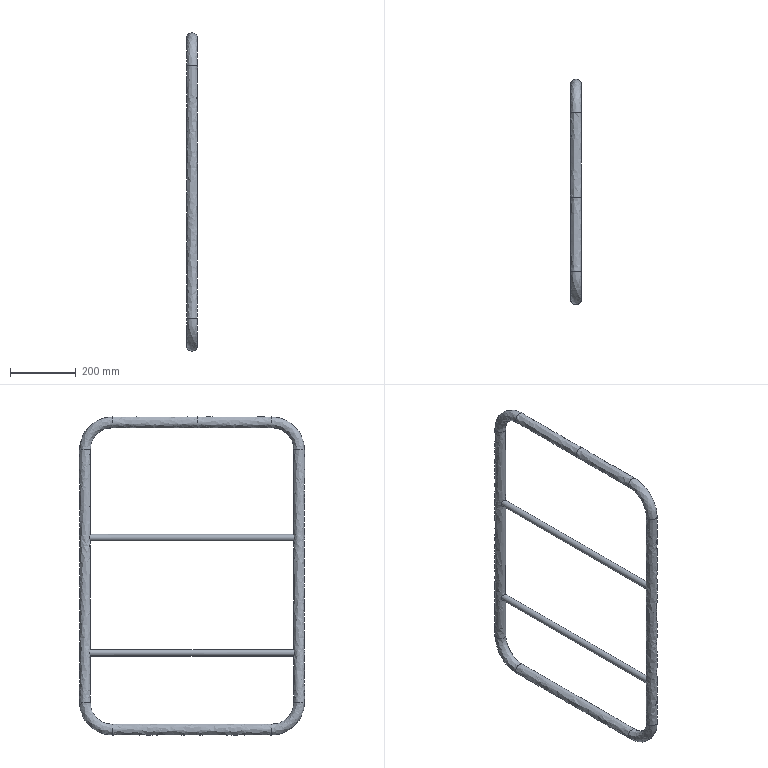Component | NX | 43_6_1 | 1 solid | 11 faces | volume 3515577 mm3 | spline 9 | cylinder 2 | commonest cylinder face diameters 20 x2